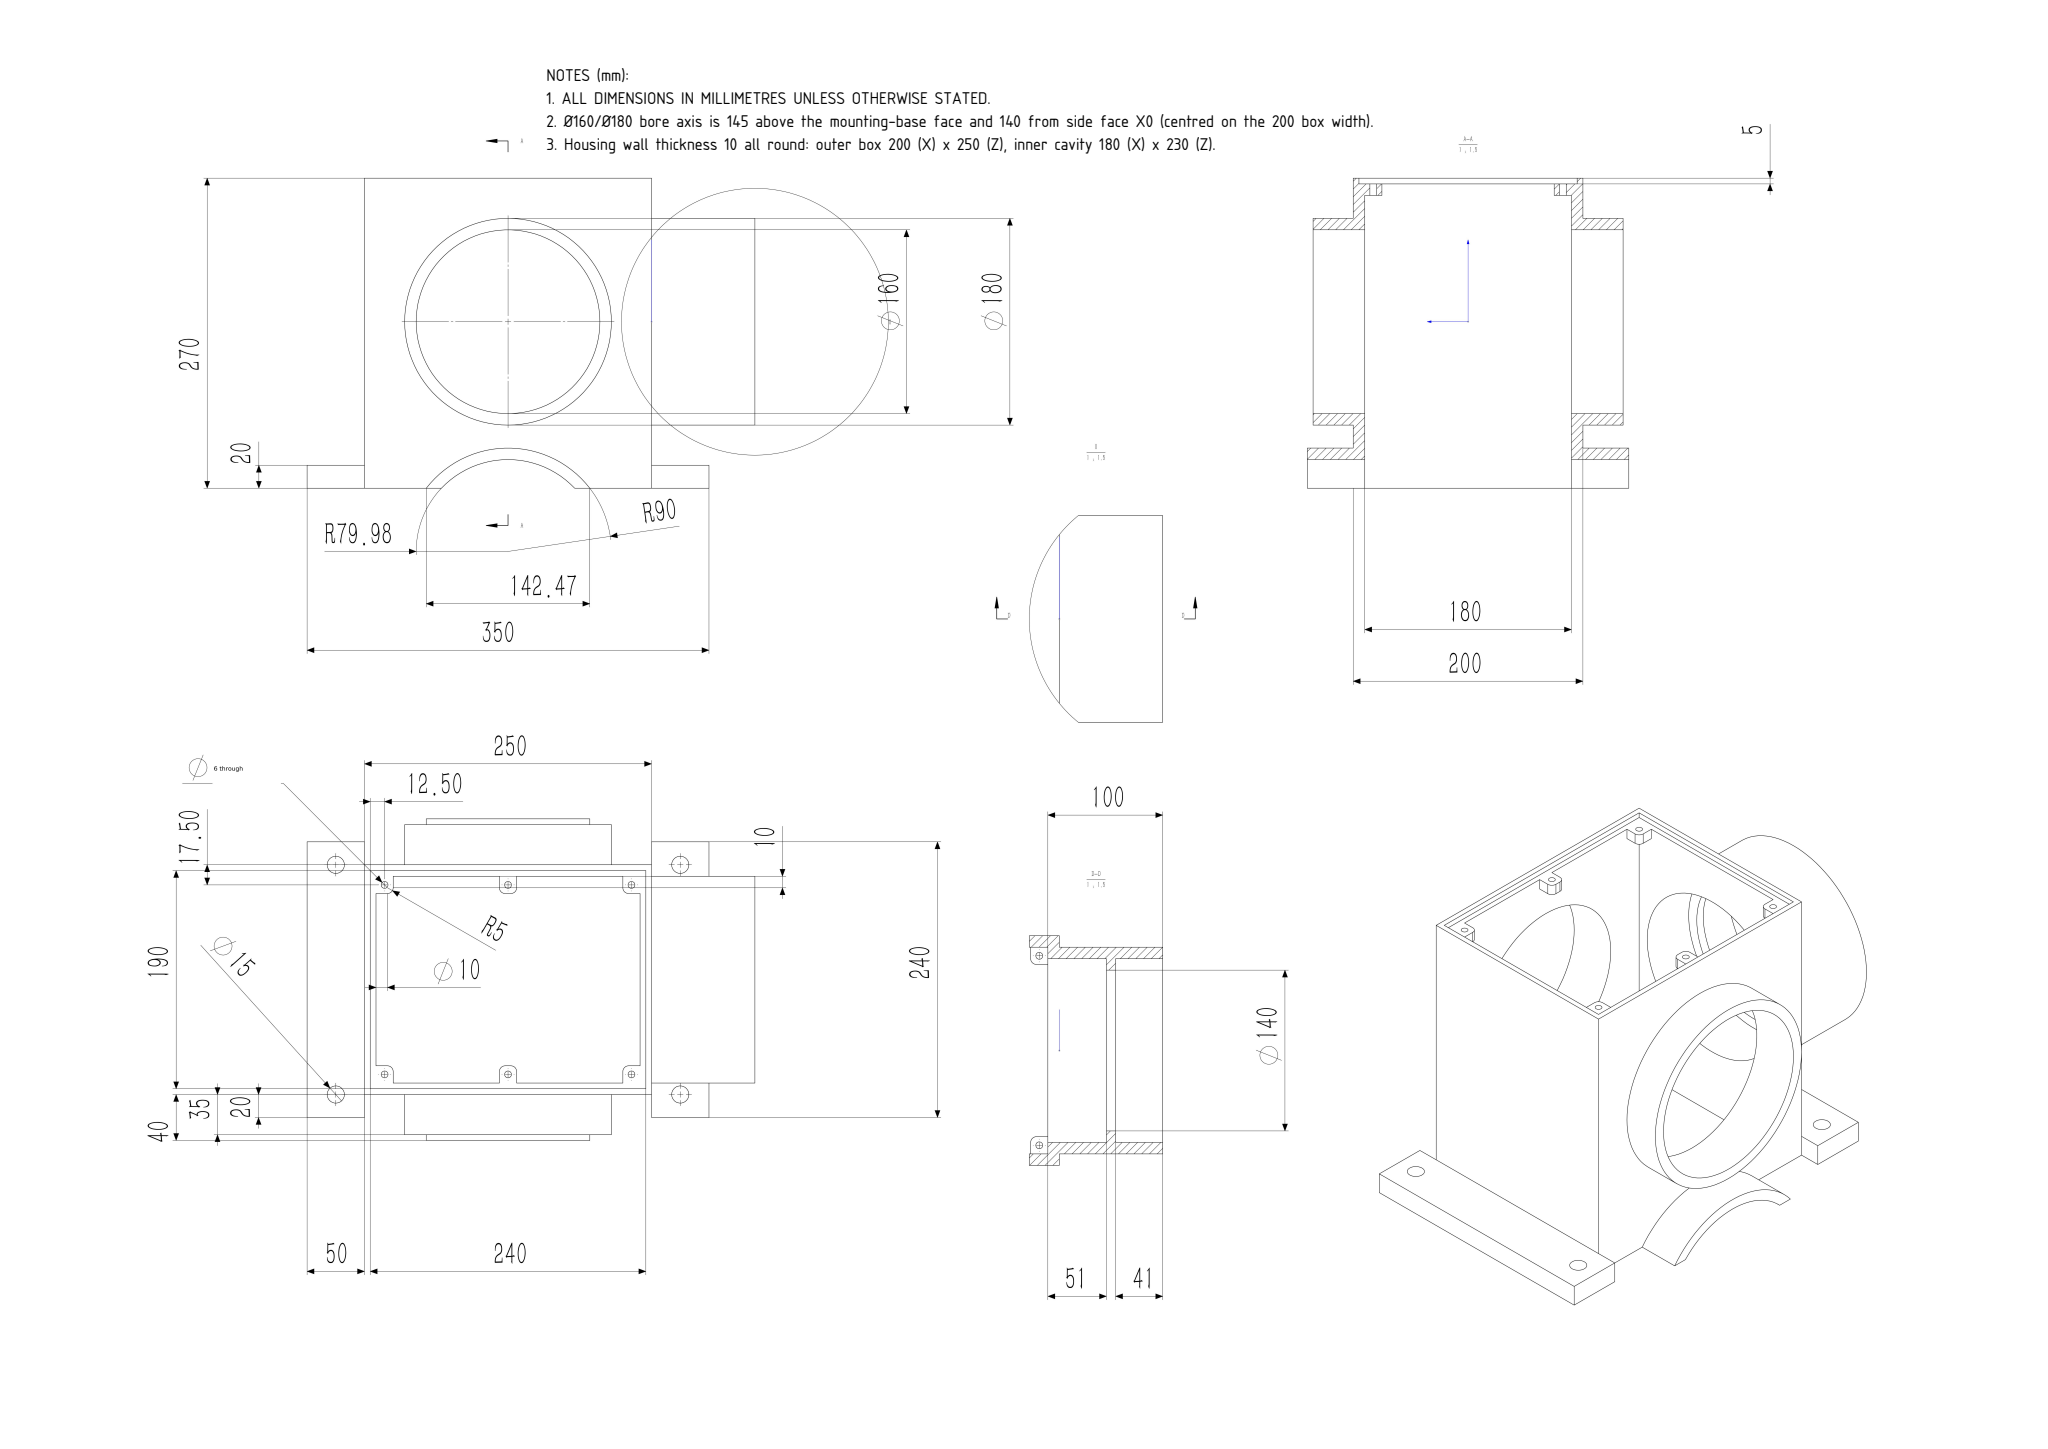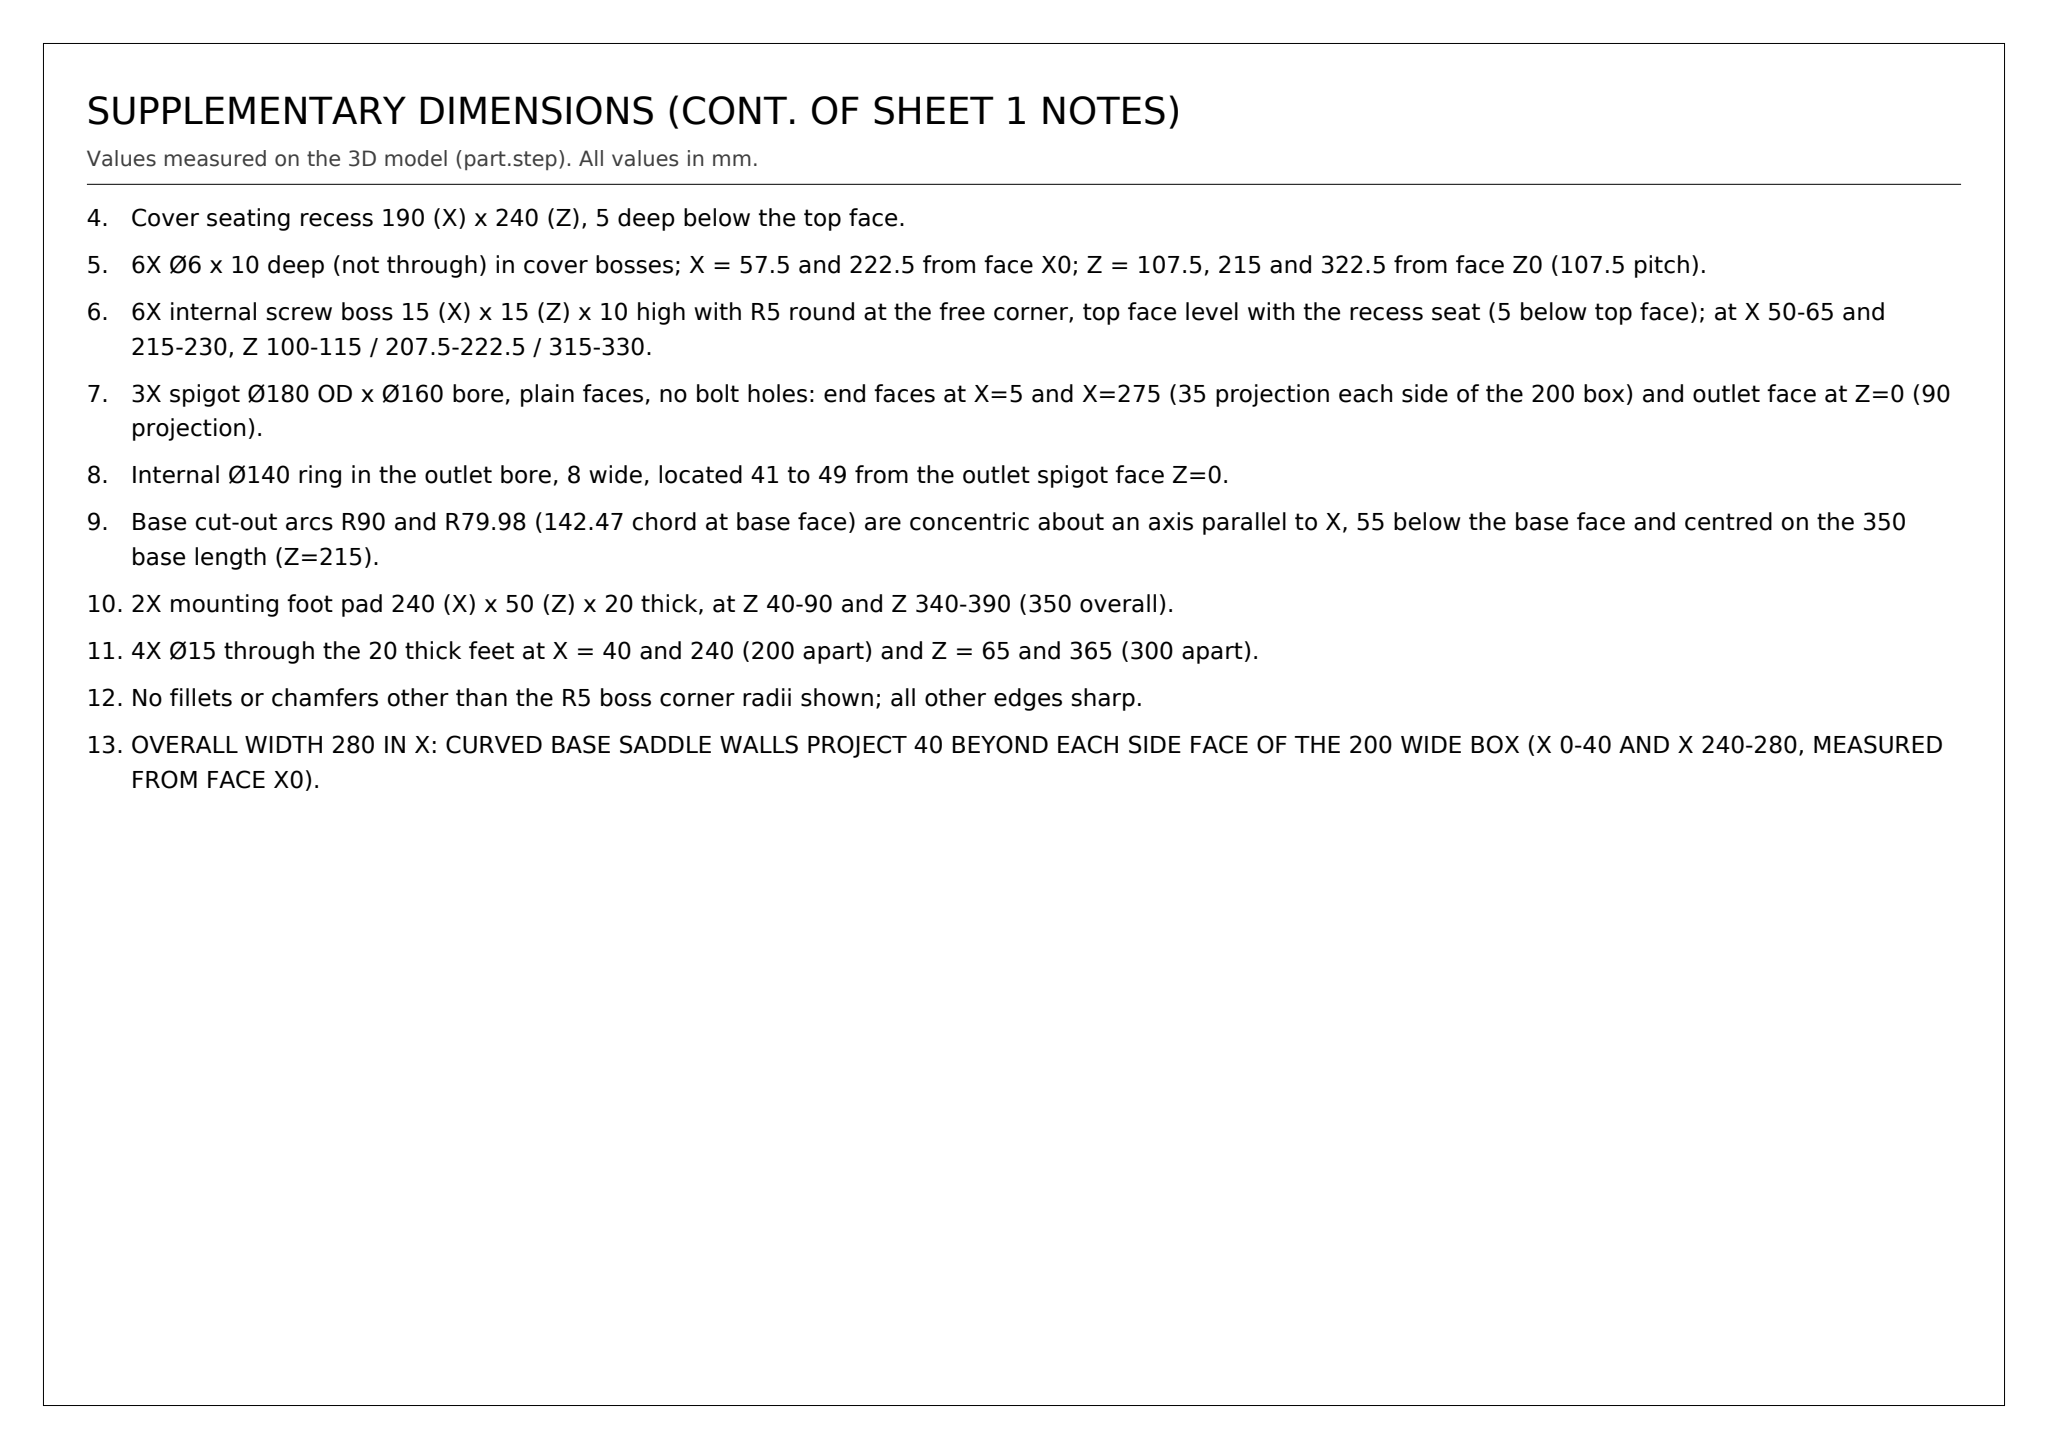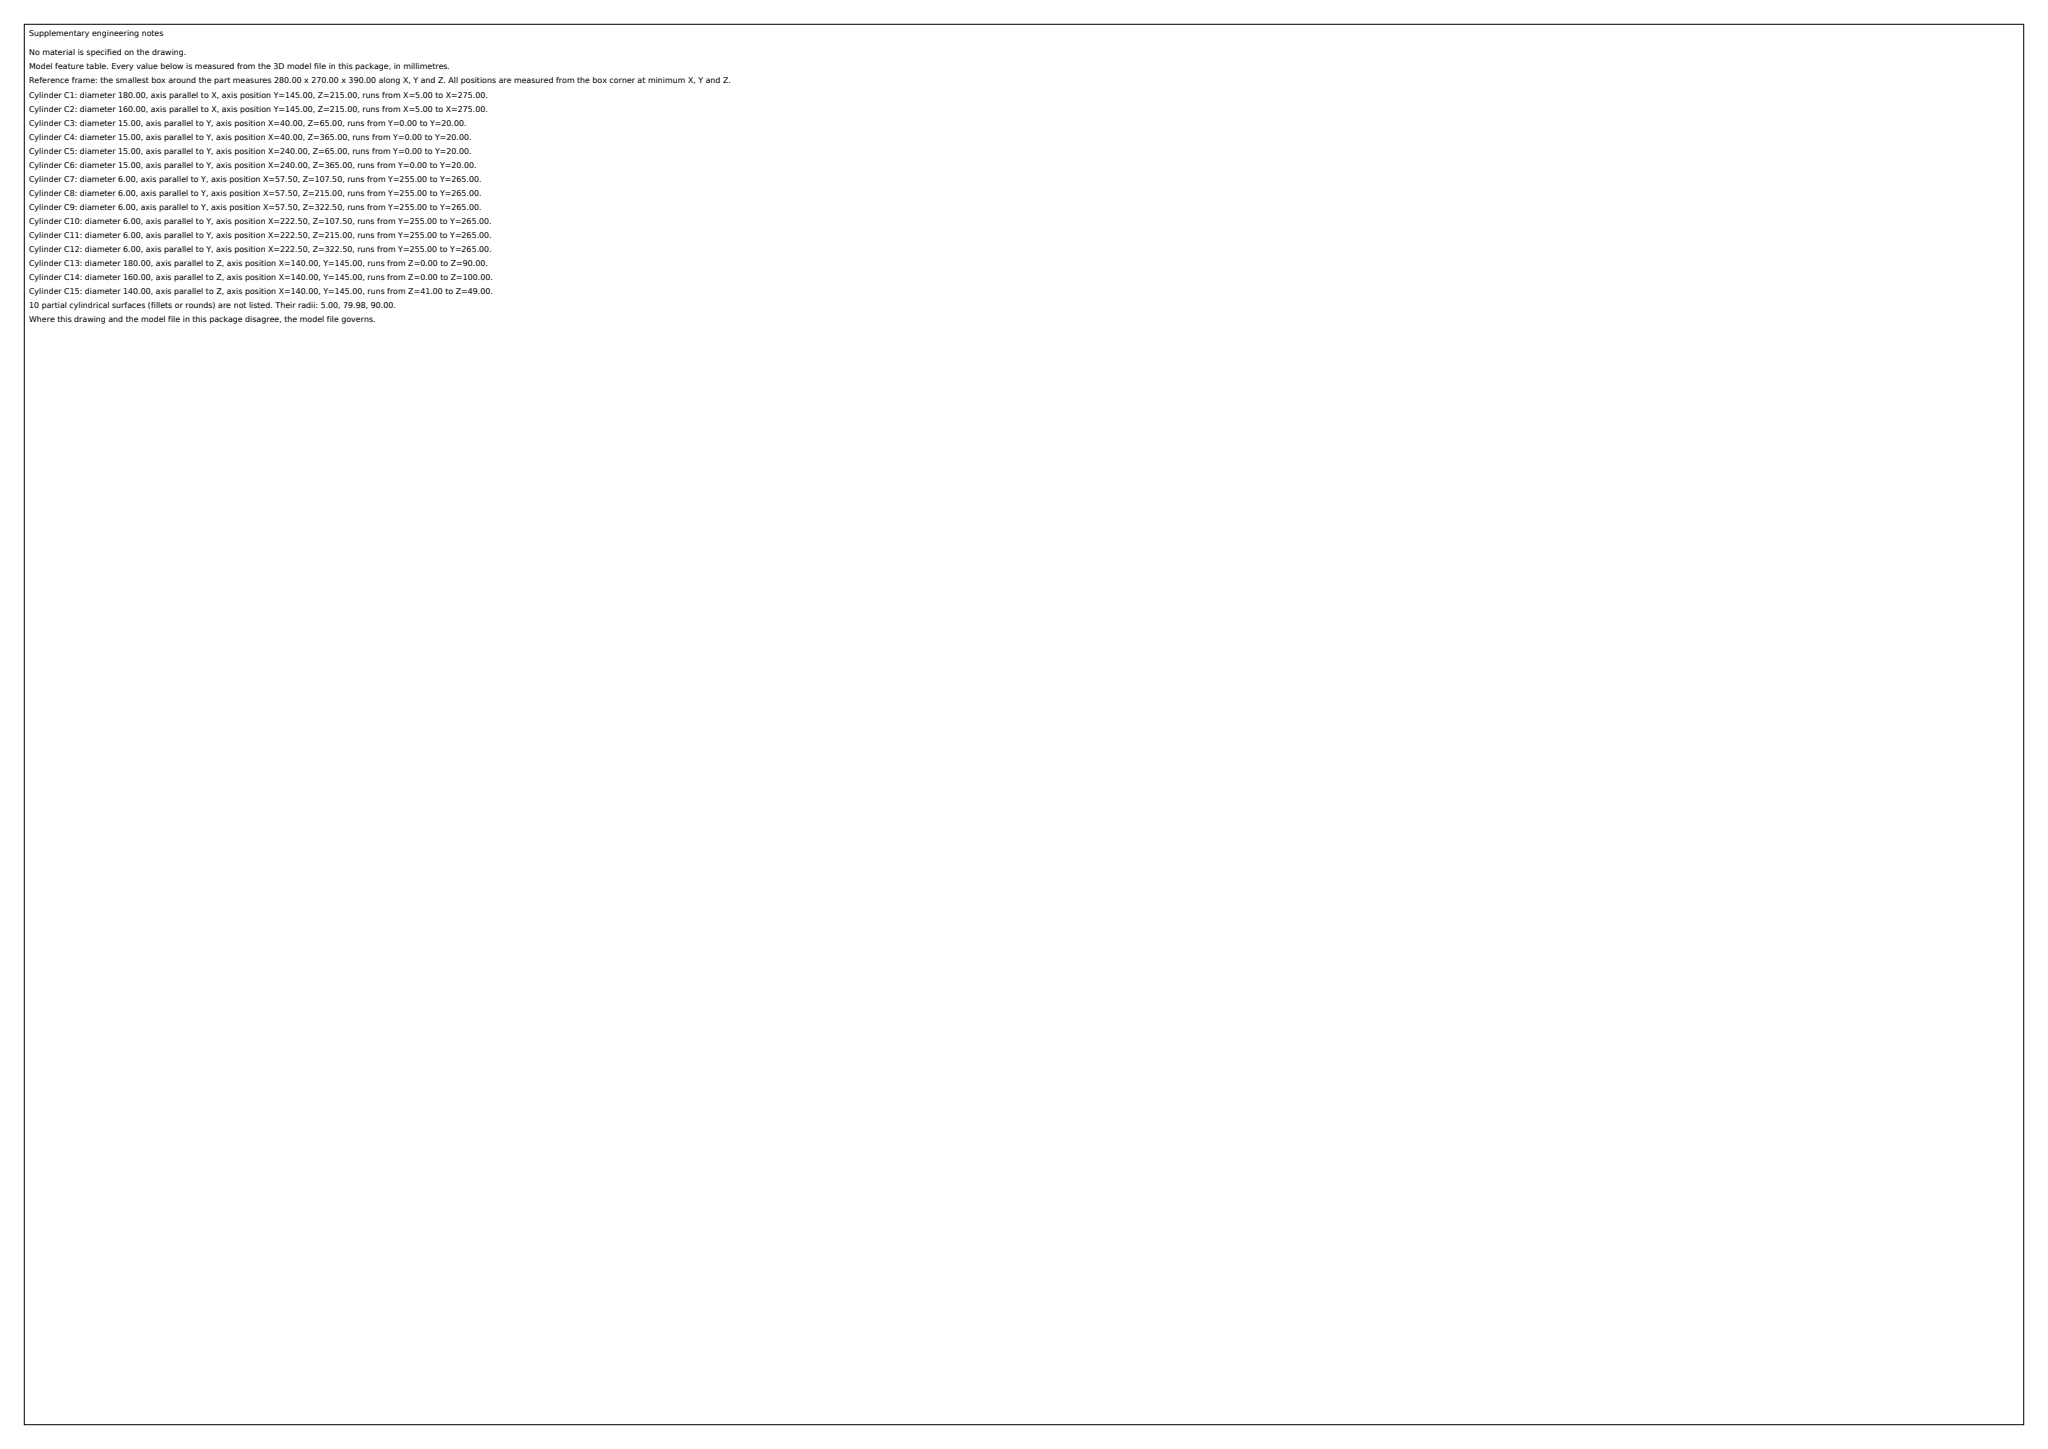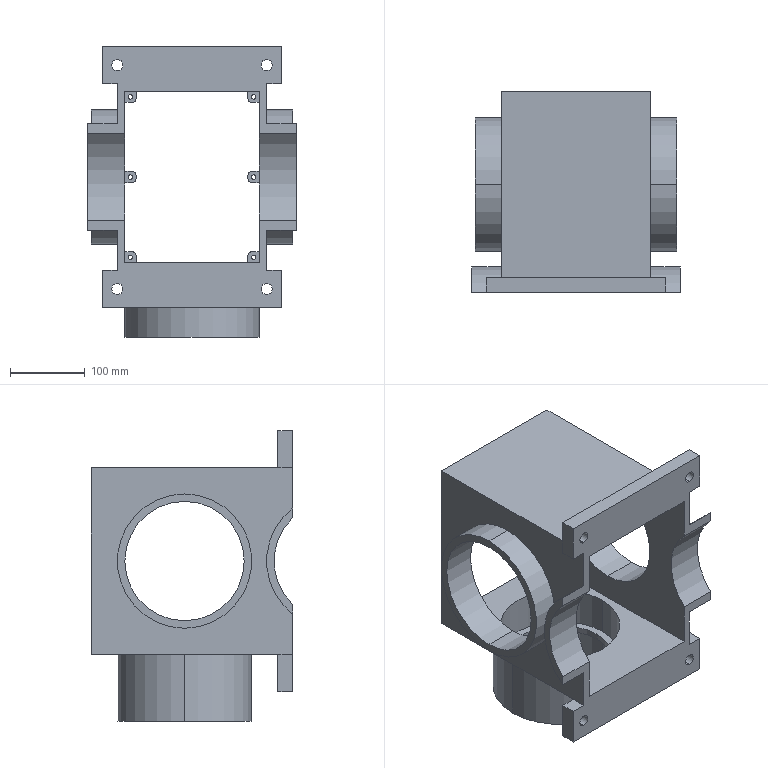Part | SolidWorks | mm | 1 solid | 103 faces | box 280 x 270 x 390 mm | volume 3145249 mm3 | plane 55 | cylinder 48 | commonest cylinder face diameters 6 x12 15 x8 160 x8 10 x8 180 x6 140 x2 159.954 x2 179.991 x2
Drawing notes:
ALL DIMENSIONS IN MILLIMETRES UNLESS OTHERWISE STATED. | from the solid: STEP model facts header: units mm
Ø160/Ø180 bore axis is 145 above the mounting-base face and 140 from side face X0 (centred on the 200 box width). | from the solid: cylinders: hole/bore 160 & boss 180, axis x, axis_pos (y=145, z=215); box outer x 40-240
Housing wall thickness 10 all round: outer box 200 (X) x 250 (Z), inner cavity 180 (X) x 230 (Z). | from the solid: planes x=40/x=240 vs x=50/x=230; planes z=90/z=340 vs z=100/z=330
Cover seating recess 190 (X) x 240 (Z), 5 deep below the top face. | from the solid: plane y=270 (x 40-240, z 90-340) and plane y=265 (x 45-235, z 95-335)
6X Ø6 x 10 deep (not through) in cover bosses; X = 57.5 and 222.5 from face X0; Z = 107.5, 215 and 322.5 from face Z0 (107.5 pitch). | from the solid: cylinders hole/bore 6.0, axis y, at (57.5/222.5, 107.5/215/322.5), from y 255 to 265
6X internal screw boss 15 (X) x 15 (Z) x 10 high with R5 round at the free corner, top face level with the recess seat (5 below top face); at X 50-65 and 215-230, Z 100-115 / 207.5-222.5 / 315-330. | from the solid: Boss base faces at y=255 span x[50,65] and x[215,230] with z[100,115] / [207.5,222.5] / [315,330] (15 x 15 footprint); boss side faces x=65 and x=215 with y[255,265] give 10 high (top at y=265 = recess seat, 5 below top face y=270); convex arcs dia 10 (R5) about y at (60,110), (60,212.5), (60,217.5), (60,320), (220,110), (220,212.5), (220,217.5), (220,320).
3X spigot Ø180 OD x Ø160 bore, plain faces, no bolt holes: end faces at X=5 and X=275 (35 projection each side of the 200 box) and outlet face at Z=0 (90 projection). | from the solid: planes x=5 and x=275 annulus area 5341 (y 55-235, z 125-305); plane z=0 annulus area 5341; boss 180 axis z from 0 to 90
Internal Ø140 ring in the outlet bore, 8 wide, located 41 to 49 from the outlet spigot face Z=0. | from the solid: hole/bore 140.0, axis z, from 41.0 to 49.0; planes z=41 and z=49, area 4712
Base cut-out arcs R90 and R79.98 (142.47 chord at base face) are concentric about an axis parallel to X, 55 below the base face and centred on the 350 base length (Z=215). | from the solid: concave arc 159.95 and convex arc 179.99, axis x, axis_pos (y=-55, z=215); plane y=0 extents z 40-156.9 and 273.1-390
2X mounting foot pad 240 (X) x 50 (Z) x 20 thick, at Z 40-90 and Z 340-390 (350 overall). | from the solid: planes y=0 / y=20 / z=40 / z=90 / z=340 / z=390 with x 20-260, y 0-20
4X Ø15 through the 20 thick feet at X = 40 and 240 (200 apart) and Z = 65 and 365 (300 apart). | from the solid: cylinders hole/bore 15.0, axis y, at (40/240, 65/365), from y 0 to 20
No fillets or chamfers other than the R5 boss corner radii shown; all other edges sharp. | from the solid: inclined_planes: empty; tori: empty; only convex arcs dia 10 (R5) at bosses
OVERALL WIDTH 280 IN X: CURVED BASE SADDLE WALLS PROJECT 40 BEYOND EACH SIDE FACE OF THE 200 WIDE BOX (X 0-40 AND X 240-280, MEASURED FROM FACE X0). | from the solid: bbox_xyz X = 280.0; axis_planes x=0.0 and x=280.0 (y 0-35, z 143.8-286.2); box side faces at x=40.0 and x=240.0
build123d program:
from build123d import *

# Parameters (mm, degrees)
SKETCH1_W               = 200
SKETCH1_H               = 250
BOSS_EXTRUDE1_DEPTH     = 250
SHELL1_T                = -10
SKETCH3_W               = 190
SKETCH3_H               = 240
SKETCH3_W_2             = 180
SKETCH3_H_2             = 230
CUT_EXTRUDE2_DEPTH      = 5
BOSS_EXTRUDE2_START     = -5
SKETCH5_R               = 3
BOSS_EXTRUDE2_DEPTH     = 10
SKETCH6_W               = 180
SKETCH6_H               = 230
CUT_EXTRUDE3_DEPTH      = 135
SKETCH7_2_R             = 90
SKETCH7_2_R_2           = 80
BOSS_EXTRUDE3_DEPTH     = 90
CUT_EXTRUDE4_START      = 80
SKETCH7_2_2_R           = 80
CUT_EXTRUDE4_DEPTH      = 80
BOSS_EXTRUDE4_START     = -41
SKETCH8_R               = 80
SKETCH8_R_2             = 70
BOSS_EXTRUDE4_DEPTH     = 8
BOSS_EXTRUDE5_START     = 100
SKETCH9_2_R             = 90
SKETCH9_2_R_2           = 80
BOSS_EXTRUDE5_DEPTH     = 35
SKETCH9_2_2_R           = 80
CUT_EXTRUDE5_DEPTH      = 117
SKETCH10_W              = 240
SKETCH10_H              = 350
SKETCH10_W_2            = 180
SKETCH10_H_2            = 230
BOSS_EXTRUDE6_DEPTH     = 20
SKETCH11_R              = 7.5
CUT_EXTRUDE6_DEPTH      = 20
MIRROR4_COPY_1_SKETCH_R = 7.5
MIRROR4_COPY_1_DEPTH    = 20
CUT_EXTRUDE7_START      = -110
SKETCH12_W              = 20
SKETCH12_H              = 250
CUT_EXTRUDE7_DEPTH      = 40
BOSS_EXTRUDE7_START     = 100
BOSS_EXTRUDE7_DEPTH     = 40
CUT_EXTRUDE9_DEPTH      = 100


with BuildPart() as part:
    # Sketch1 → Boss-Extrude1 (new body)
    with BuildSketch(Plane.XY):
        Rectangle(SKETCH1_W, SKETCH1_H)
    extrude(amount=BOSS_EXTRUDE1_DEPTH)

    # Shell1
    shell1_openings = [part.faces().sort_by_distance(p)[0] for p in [
        (0, 125, 125),
    ]]
    offset(amount=SHELL1_T, openings=shell1_openings, kind=Kind.INTERSECTION)

    # Sketch3 → Cut-Extrude2 (cut)
    with BuildSketch(Plane(origin=(0, 125, 0), x_dir=(1, 0, 0), z_dir=(0, 1, 0))):
        with Locations((0, -125)):
            Rectangle(SKETCH3_W, SKETCH3_H)
        with Locations((0, -125)):
            Rectangle(SKETCH3_W_2, SKETCH3_H_2, mode=Mode.SUBTRACT)
    extrude(amount=-CUT_EXTRUDE2_DEPTH, mode=Mode.SUBTRACT)

    # Sketch5 → Boss-Extrude2 (add)
    # profile 1 of 3: a face of its own
    with BuildSketch(Plane(origin=(0, 125, 0), x_dir=(1, 0, 0), z_dir=(0, 1, 0)).offset(BOSS_EXTRUDE2_START)):
        with BuildLine():
            Line((-90, -10), (-75, -10))
            Line((-75, -10), (-75, -20))
            ThreePointArc((-75, -20), (-76.464, -23.536), (-80, -25))
            Line((-80, -25), (-90, -25))
            Line((-90, -25), (-90, -10))
        make_face()
        with Locations(Location((-82.5, -17.5, 0), (0, 0, 270))):
            Circle(SKETCH5_R, mode=Mode.SUBTRACT)
    # profile 2 of 3: a face of its own
    with BuildSketch(Plane(origin=(0, 125, 0), x_dir=(1, 0, 0), z_dir=(0, 1, 0)).offset(BOSS_EXTRUDE2_START)):
        with BuildLine():
            Line((-90, -125), (-90, -117.5))
            Line((-90, -117.5), (-80, -117.5))
            ThreePointArc((-80, -117.5), (-76.464, -118.964), (-75, -122.5))
            Line((-75, -122.5), (-75, -127.5))
            ThreePointArc((-75, -127.5), (-76.464, -131.036), (-80, -132.5))
            Line((-80, -132.5), (-90, -132.5))
            Line((-90, -132.5), (-90, -125))
        make_face()
        with Locations(Location((-82.5, -125, 0), (0, 0, 270))):
            Circle(SKETCH5_R, mode=Mode.SUBTRACT)
    # profile 3 of 3: a face of its own
    with BuildSketch(Plane(origin=(0, 125, 0), x_dir=(1, 0, 0), z_dir=(0, 1, 0)).offset(BOSS_EXTRUDE2_START)):
        with BuildLine():
            Line((-90, -240), (-90, -225))
            Line((-90, -225), (-80, -225))
            ThreePointArc((-80, -225), (-76.464, -226.464), (-75, -230))
            Line((-75, -230), (-75, -240))
            Line((-75, -240), (-90, -240))
        make_face()
        with Locations(Location((-82.5, -232.5, 0), (0, 0, 270))):
            Circle(SKETCH5_R, mode=Mode.SUBTRACT)
    boss_extrude2 = extrude(amount=-BOSS_EXTRUDE2_DEPTH)

    # Mirror1: Boss-Extrude2 across plane
    add(boss_extrude2.mirror(Plane(origin=(0, 0, 0), x_dir=(0, 0, 1), z_dir=(1, 0, 0))))

    # Sketch6 → Cut-Extrude3 (cut)
    with BuildSketch(Plane(origin=(0, 0, 0), x_dir=(1, 0, 0), z_dir=(0, 1, 0))):
        with Locations((0, -125)):
            Rectangle(SKETCH6_W, SKETCH6_H)
    extrude(amount=-CUT_EXTRUDE3_DEPTH, mode=Mode.SUBTRACT)

    # Sketch7_2 → Boss-Extrude3 (add)
    with BuildSketch(Plane.XY):
        Circle(SKETCH7_2_R)
        Circle(SKETCH7_2_R_2, mode=Mode.SUBTRACT)
    extrude(amount=-BOSS_EXTRUDE3_DEPTH)

    # Sketch7_2 2 → Cut-Extrude4 (cut)
    with BuildSketch(Plane.XY.offset(CUT_EXTRUDE4_START)):
        Circle(SKETCH7_2_2_R)
    extrude(amount=-CUT_EXTRUDE4_DEPTH, mode=Mode.SUBTRACT)

    # Sketch8 → Boss-Extrude4 (add)
    with BuildSketch(Plane.XY.offset(BOSS_EXTRUDE4_START)):
        Circle(SKETCH8_R)
        Circle(SKETCH8_R_2, mode=Mode.SUBTRACT)
    extrude(amount=-BOSS_EXTRUDE4_DEPTH)

    # Sketch9_2 → Boss-Extrude5 (add)
    with BuildSketch(Plane(origin=(0, 0, 0), x_dir=(0, 0, -1), z_dir=(1, 0, 0)).offset(BOSS_EXTRUDE5_START)):
        with Locations(Location((-125, 0, 0), (0, 0, 270))):
            Circle(SKETCH9_2_R)
        with Locations((-125, 0)):
            Circle(SKETCH9_2_R_2, mode=Mode.SUBTRACT)
    boss_extrude5 = extrude(amount=BOSS_EXTRUDE5_DEPTH)

    # Sketch9_2 2 → Cut-Extrude5 (cut, symmetric)
    with BuildSketch(Plane(origin=(0, 0, 0), x_dir=(0, 0, -1), z_dir=(1, 0, 0))):
        with Locations(Location((-125, 0, 0), (0, 0, 270))):
            Circle(SKETCH9_2_2_R)
    extrude(amount=CUT_EXTRUDE5_DEPTH, both=True, mode=Mode.SUBTRACT)

    # Mirror2: Boss-Extrude5 across plane
    add(boss_extrude5.mirror(Plane(origin=(0, 0, 0), x_dir=(0, 0, 1), z_dir=(1, 0, 0))))



with BuildPart() as body_2:
    # Sketch10 → Boss-Extrude6 (new body)
    with BuildSketch(Plane(origin=(0, -125, 0), x_dir=(-1, 0, 0), z_dir=(0, -1, 0))):
        with Locations((0, -125)):
            Rectangle(SKETCH10_W, SKETCH10_H)
        with Locations((0, -125)):
            Rectangle(SKETCH10_W_2, SKETCH10_H_2, mode=Mode.SUBTRACT)
    extrude(amount=BOSS_EXTRUDE6_DEPTH)

    # Sketch11 → Cut-Extrude6 (cut)
    with BuildSketch(Plane(origin=(0, -125, 0), x_dir=(-1, 0, 0), z_dir=(0, -1, 0))):
        with Locations(Location((-100, -275, 0), (0, 0, 90))):
            Circle(SKETCH11_R)
    cut_extrude6 = extrude(amount=CUT_EXTRUDE6_DEPTH, mode=Mode.SUBTRACT)

    # Mirror3: Cut-Extrude6 across plane
    add(cut_extrude6.mirror(Plane(origin=(0, 0, 0), x_dir=(0, 0, 1), z_dir=(1, 0, 0))), mode=Mode.SUBTRACT)

    # Mirror4: Cut-Extrude6 across plane
    add(cut_extrude6.mirror(Plane.XY.offset(125)), mode=Mode.SUBTRACT)

    # Mirror4 copy 1 sketch → Mirror4 copy 1 (cut)
    with BuildSketch(Plane(origin=(0, -125, 250), x_dir=(1, 0, 0), z_dir=(0, -1, 0))):
        with Locations(Location((-100, -275, 0), (0, 0, 90))):
            Circle(MIRROR4_COPY_1_SKETCH_R)
    extrude(amount=MIRROR4_COPY_1_DEPTH, mode=Mode.SUBTRACT)

    # Sketch12 → Cut-Extrude7 (cut)
    with BuildSketch(Plane(origin=(0, 0, 0), x_dir=(1, 0, 0), z_dir=(0, 1, 0)).offset(CUT_EXTRUDE7_START)):
        with Locations((110, -125)):
            Rectangle(SKETCH12_W, SKETCH12_H)
        with Locations((-110, -125)):
            Rectangle(SKETCH12_W, SKETCH12_H)
    extrude(amount=-CUT_EXTRUDE7_DEPTH, mode=Mode.SUBTRACT)


with BuildPart() as part_1:
    add(part.part)

    add(body_2.part)  # Boss-Extrude7 merges body 2
    # Sketch13_5 → Boss-Extrude7 (add)
    with BuildSketch(Plane(origin=(0, 0, 0), x_dir=(0, 0, -1), z_dir=(1, 0, 0)).offset(BOSS_EXTRUDE7_START)):
        with BuildLine():
            Line((-125, -120.023), (-125, -110.004))
            ThreePointArc((-125, -110.004), (-164.683, -119.226), (-196.233, -145))
            Line((-196.233, -145), (-183.063, -145))
            ThreePointArc((-183.063, -145), (-156.604, -126.532), (-125, -120.023))
        make_face()
        with BuildLine():
            ThreePointArc((-53.767, -145), (-85.317, -119.226), (-125, -110.004))
            Line((-125, -110.004), (-125, -120.023))
            ThreePointArc((-125, -120.023), (-93.396, -126.532), (-66.937, -145))
            Line((-66.937, -145), (-53.767, -145))
        make_face()
    boss_extrude7 = extrude(amount=BOSS_EXTRUDE7_DEPTH)

    # Sketch13_5 2 → Cut-Extrude9 (cut, symmetric)
    with BuildSketch(Plane(origin=(0, 0, 0), x_dir=(0, 0, -1), z_dir=(1, 0, 0))):
        with BuildLine():
            ThreePointArc((-66.937, -145), (-93.396, -126.532), (-125, -120.023))
            Line((-125, -120.023), (-125, -145))
            Line((-125, -145), (-66.937, -145))
        make_face()
        with BuildLine():
            Line((-125, -145), (-125, -120.023))
            ThreePointArc((-125, -120.023), (-156.604, -126.532), (-183.063, -145))
            Line((-183.063, -145), (-125, -145))
        make_face()
        with BuildLine():
            ThreePointArc((-66.937, -145), (-93.396, -126.532), (-125, -120.023))
            Line((-125, -120.023), (-125, -145))
            Line((-125, -145), (-66.937, -145))
        make_face()
        with BuildLine():
            Line((-125, -145), (-125, -120.023))
            ThreePointArc((-125, -120.023), (-156.604, -126.532), (-183.063, -145))
            Line((-183.063, -145), (-125, -145))
        make_face()
    extrude(amount=CUT_EXTRUDE9_DEPTH, both=True, mode=Mode.SUBTRACT)

    # Mirror5: Boss-Extrude7 across plane
    add(boss_extrude7.mirror(Plane(origin=(0, 0, 0), x_dir=(0, 0, 1), z_dir=(1, 0, 0))))


solid = part_1.part